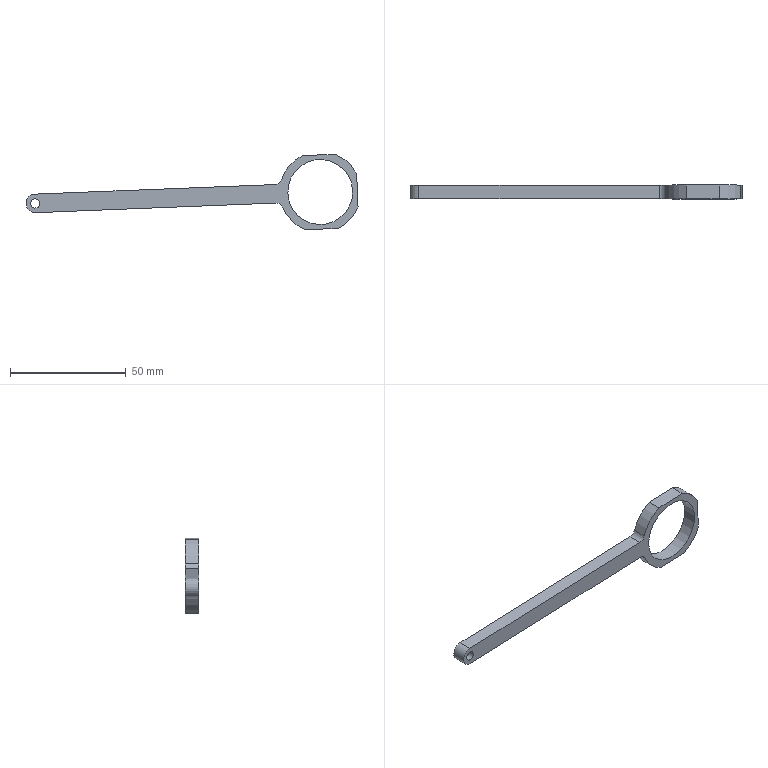Component | NX | CONNECTING_ROD_2_2 | 1 solid | 16 faces | volume 6978 mm3 | cylinder 9 | plane 7 | commonest cylinder face diameters 35 x4 6 x2 8 x1 28 x1 4 x1